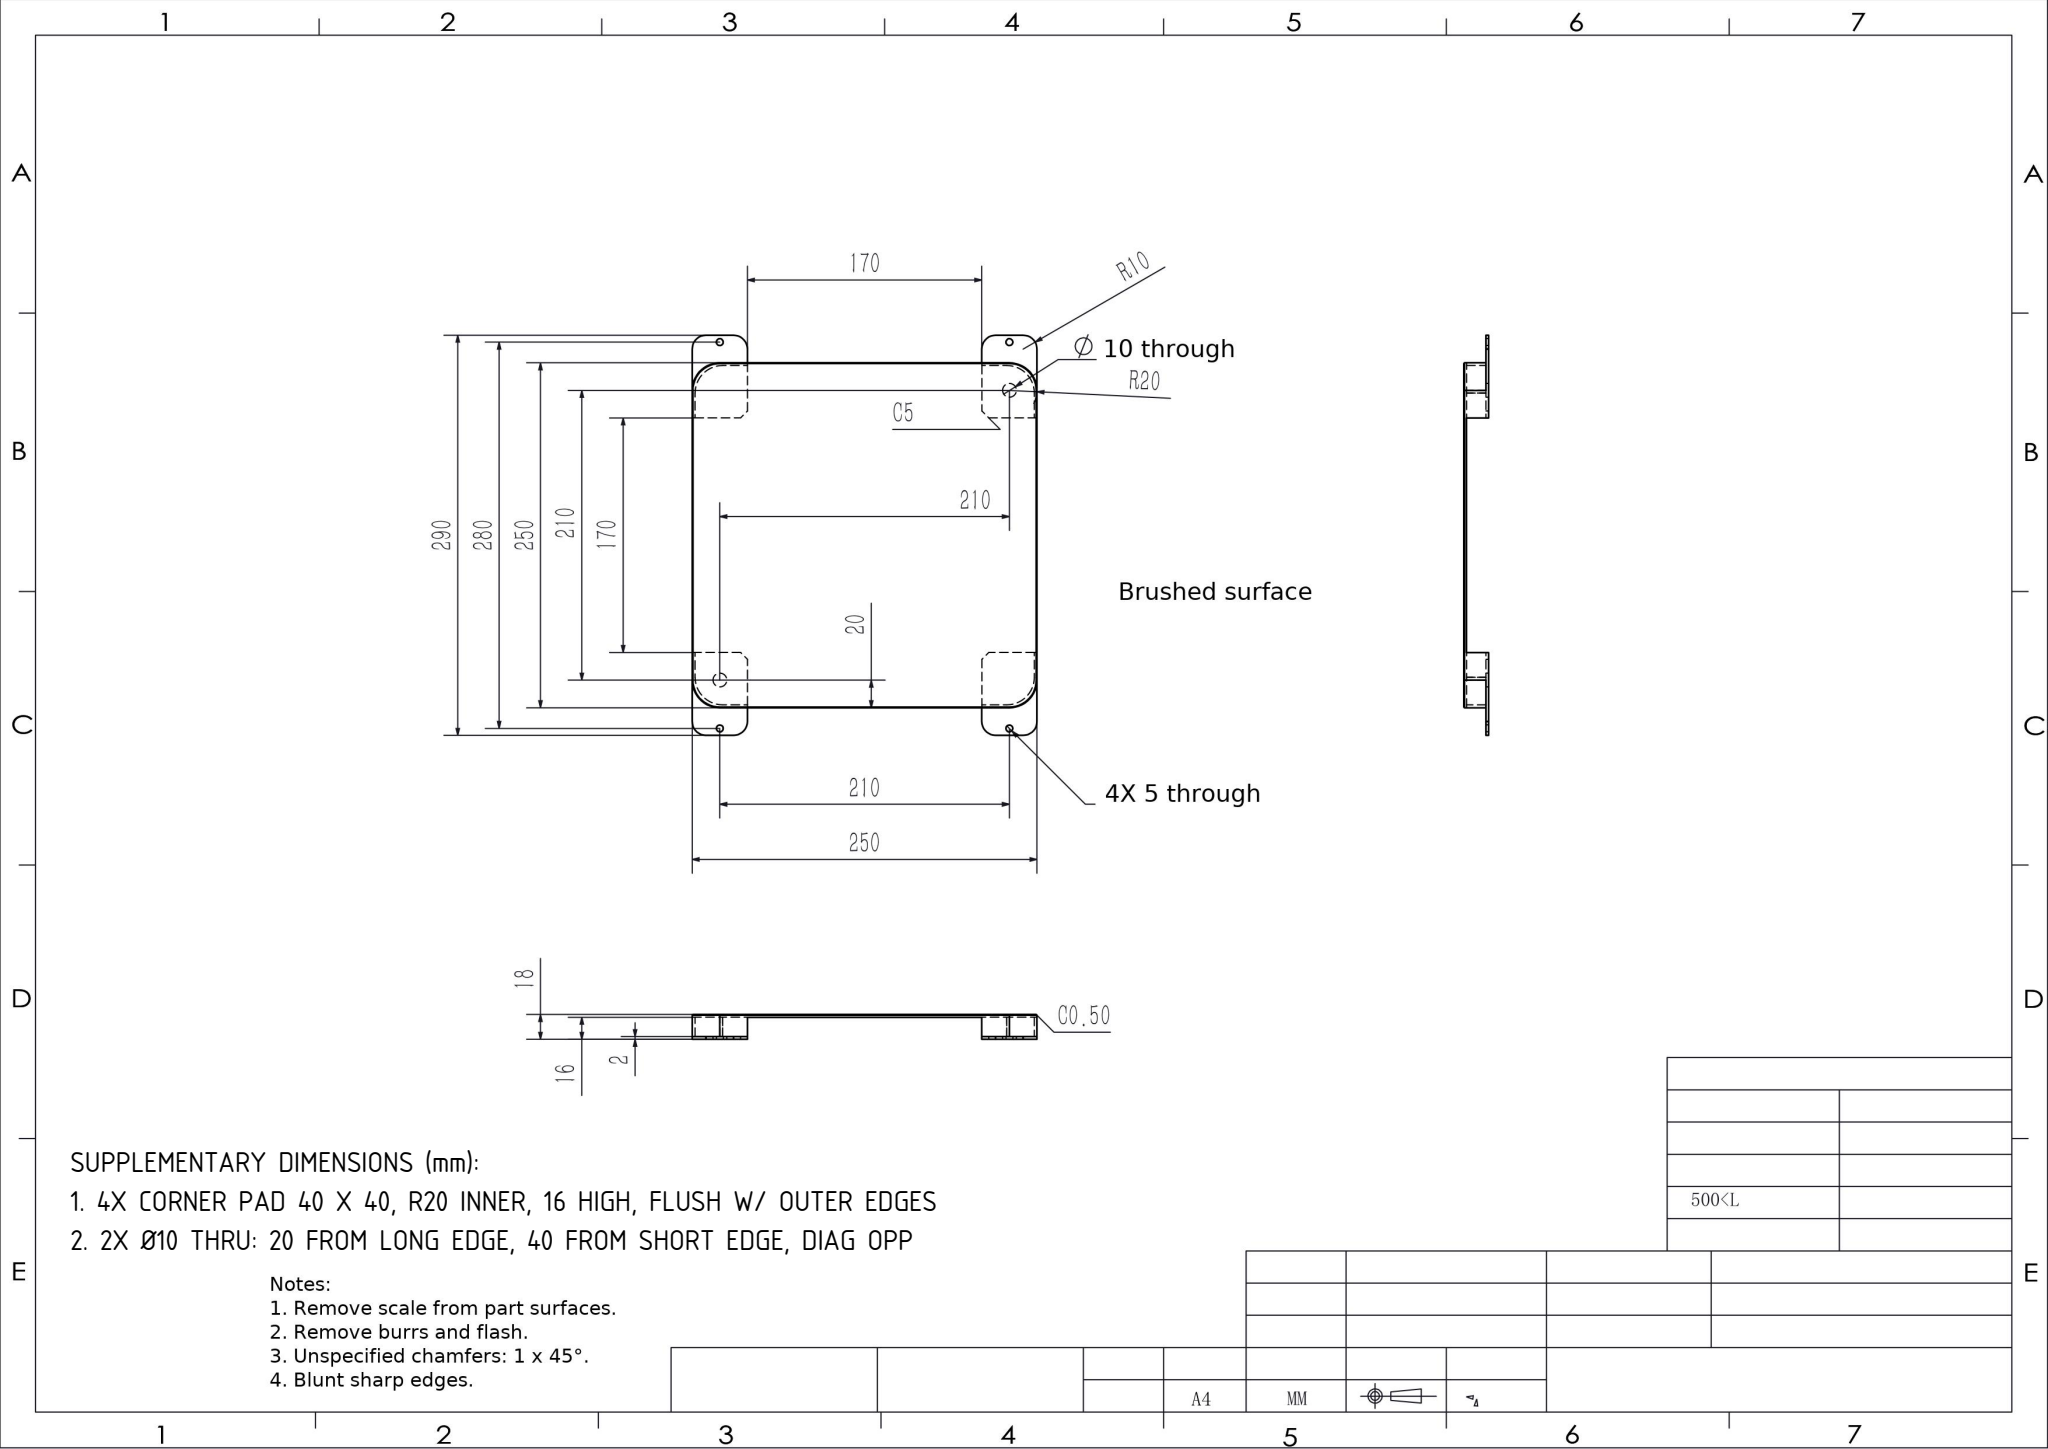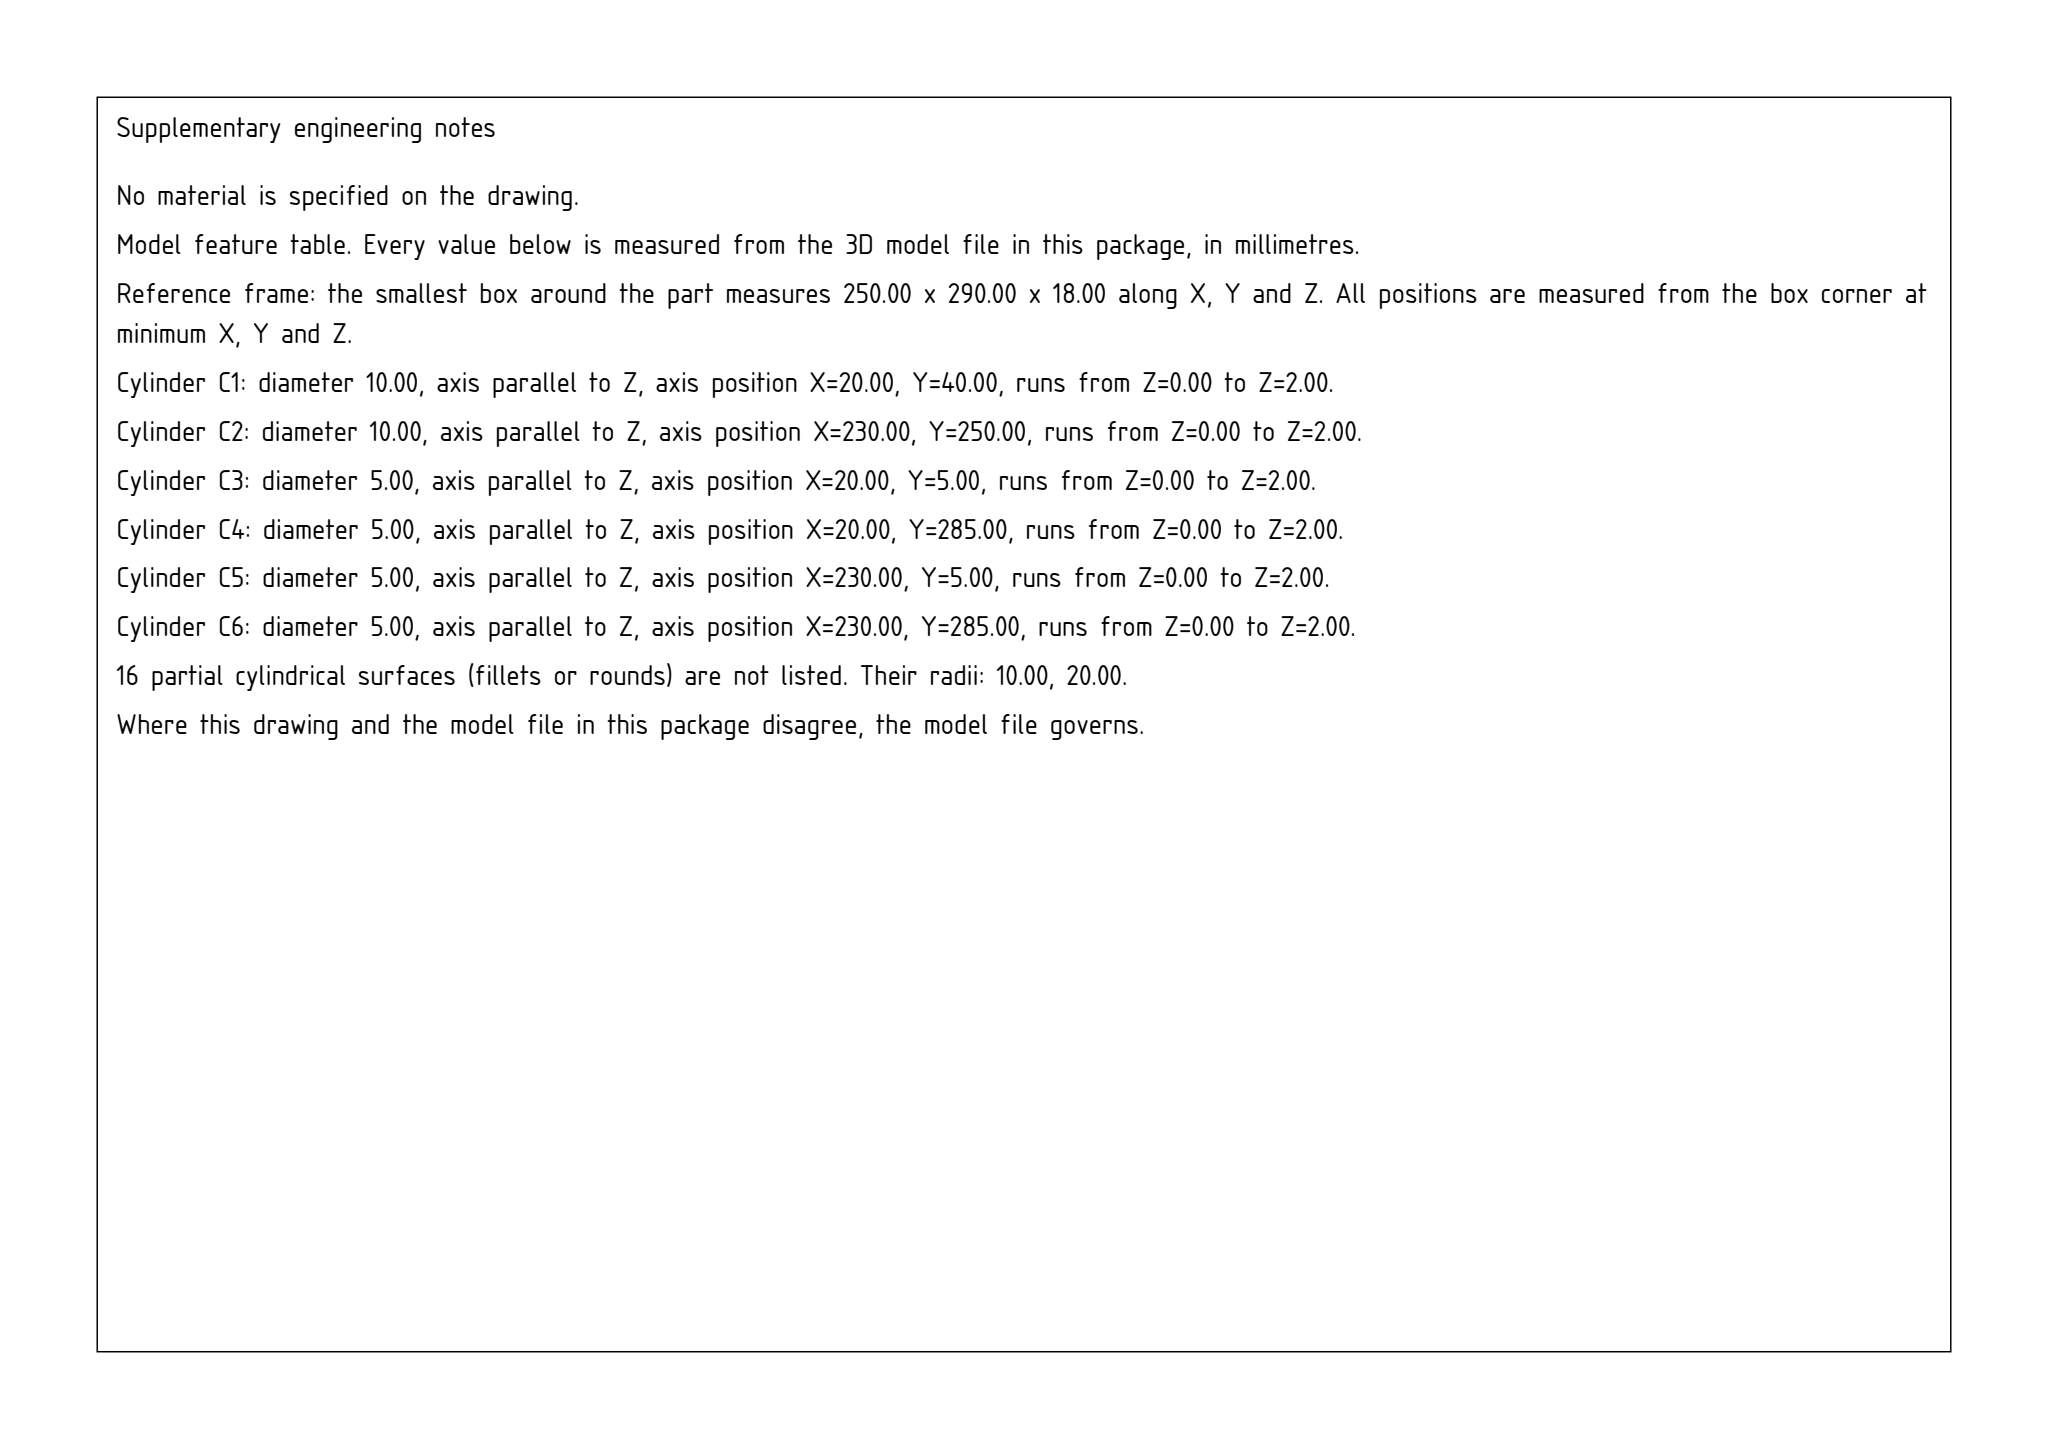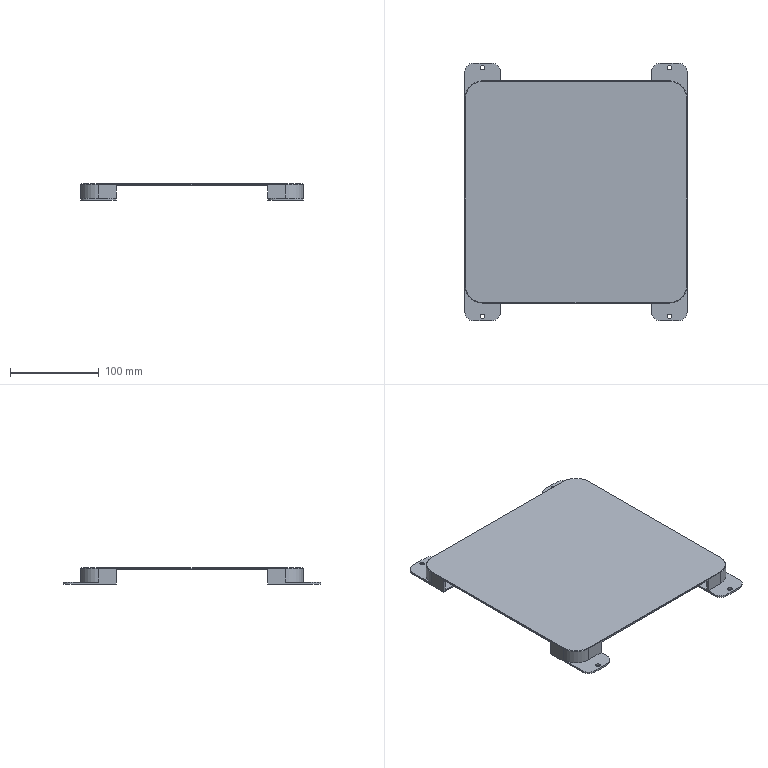Part | SolidWorks | mm | 1 solid | 78 faces | box 250 x 290 x 18 mm | volume 151214 mm3 | plane 46 | cylinder 28 | cone 4 | commonest cylinder face diameters 5 x8 40 x8 20 x8 10 x4
build123d program:
from build123d import *

# Parameters (mm, degrees)
SKETCH1_W           = 250
SKETCH1_H           = 250
BOSS_EXTRUDE1_DEPTH = 2
BOSS_EXTRUDE2_DEPTH = 14
SKETCH5_W           = 40
SKETCH5_H           = 40
BOSS_EXTRUDE3_DEPTH = 2
FILLET1_R           = 20
FILLET2_R           = 20
CHAMFER1_SIZE       = 0.5
CHAMFER2_SIZE       = 5
SKETCH6_R           = 5
CUT_EXTRUDE1_DEPTH  = 2
BOSS_EXTRUDE4_DEPTH = 2
FILLET3_R           = 10
SKETCH9_R           = 2.5
CUT_EXTRUDE2_DEPTH  = 193.109


with BuildPart() as part:
    # Sketch1 → Boss-Extrude1 (new body)
    with BuildSketch(Plane.XY):
        Rectangle(SKETCH1_W, SKETCH1_H)
    extrude(amount=BOSS_EXTRUDE1_DEPTH)

    # Sketch4 → Boss-Extrude2 (add)
    with BuildSketch(Plane(origin=(0, 0, 0), x_dir=(-1, 0, 0), z_dir=(0, 0, -1))):
        Polygon((85, 125), (125, 125), (125, 85), (123, 85), (123, 123), (85, 123), align=None)
        Polygon((-85, 123), (-123, 123), (-123, 85), (-125, 85), (-125, 125), (-85, 125), align=None)
        Polygon((-85, -125), (-125, -125), (-125, -85), (-123, -85), (-123, -123), (-85, -123), align=None)
        Polygon((85, -123), (123, -123), (123, -85), (125, -85), (125, -125), (85, -125), align=None)
    extrude(amount=BOSS_EXTRUDE2_DEPTH)

    # Sketch5 → Boss-Extrude3 (add)
    with BuildSketch(Plane(origin=(0, 0, -14), x_dir=(-1, 0, 0), z_dir=(0, 0, -1))):
        with Locations((105, 105)):
            Rectangle(SKETCH5_W, SKETCH5_H)
        with Locations((105, -105)):
            Rectangle(SKETCH5_W, SKETCH5_H)
        with Locations((-105, -105)):
            Rectangle(SKETCH5_W, SKETCH5_H)
        with Locations((-105, 105)):
            Rectangle(SKETCH5_W, SKETCH5_H)
    extrude(amount=BOSS_EXTRUDE3_DEPTH)

    # Fillet1
    fillet1_edges = [part.edges().sort_by_distance(p)[0] for p in [
        (125, -125, -7),
        (-125, -125, -7),
        (-125, 125, -7),
        (125, 125, -7),
    ]]
    fillet(fillet1_edges, radius=FILLET1_R)

    # Fillet2
    fillet2_edges = [part.edges().sort_by_distance(p)[0] for p in [
        (-123, 123, -7),
        (123, 123, -7),
        (123, -123, -7),
        (-123, -123, -7),
    ]]
    fillet(fillet2_edges, radius=FILLET2_R)

    # Chamfer1
    chamfer1_edges = [part.edges().sort_by_distance(p)[0] for p in [
        (-125, 0, 2),
        (0, 125, 2),
        (125, 0, 2),
        (0, -125, 2),
        (-119.142, -119.142, 2),
        (119.142, -119.142, 2),
        (119.142, 119.142, 2),
        (-119.142, 119.142, 2),
    ]]
    chamfer(chamfer1_edges, length=CHAMFER1_SIZE)

    # Chamfer2
    chamfer2_edges = [part.edges().sort_by_distance(p)[0] for p in [
        (85, -85, -15),
        (85, 85, -15),
        (-85, 85, -15),
        (-85, -85, -15),
    ]]
    chamfer(chamfer2_edges, length=CHAMFER2_SIZE)

    # Sketch6 → Cut-Extrude1 (cut)
    with BuildSketch(Plane(origin=(0, 0, -16), x_dir=(-1, 0, 0), z_dir=(0, 0, -1))):
        with Locations((-105, 105)):
            Circle(SKETCH6_R)
        with Locations((105, -105)):
            Circle(SKETCH6_R)
    extrude(amount=-CUT_EXTRUDE1_DEPTH, mode=Mode.SUBTRACT)

    # Sketch8 → Boss-Extrude4 (add)
    with BuildSketch(Plane(origin=(0, 0, -16), x_dir=(-1, 0, 0), z_dir=(0, 0, -1))):
        Polygon((-85, -100.761), (-95.852, -100.761), (-95.852, -116.476), (-113.788, -116.476), (-113.788, -100.761), (-125, -100.761), (-125, -145), (-85, -145), align=None)
        Polygon((-95.852, 100.761), (-95.852, 116.476), (-113.788, 116.476), (-113.788, 100.761), (-125, 100.761), (-125, 145), (-85, 145), (-85, 100.761), align=None)
        Polygon((95.852, -100.761), (95.852, -116.476), (113.788, -116.476), (113.788, -100.761), (125, -100.761), (125, -145), (85, -145), (85, -100.761), align=None)
        Polygon((85, 100.761), (95.852, 100.761), (95.852, 116.476), (113.788, 116.476), (113.788, 100.761), (125, 100.761), (125, 145), (85, 145), align=None)
    extrude(amount=-BOSS_EXTRUDE4_DEPTH)

    # Fillet3
    fillet3_edges = [part.edges().sort_by_distance(p)[0] for p in [
        (85, -145, -15),
        (125, -145, -15),
        (85, 145, -15),
        (125, 145, -15),
        (-85, -145, -15),
        (-125, -145, -15),
        (-85, 145, -15),
        (-125, 145, -15),
    ]]
    fillet(fillet3_edges, radius=FILLET3_R)

    # Sketch9 → Cut-Extrude2 (cut, through all)
    with BuildSketch(Plane.XY.offset(-14)):
        with Locations((-105, 140)):
            Circle(SKETCH9_R)
        with Locations(Location((105, 140, 0), (0, 0, 180))):
            Circle(SKETCH9_R)
        with Locations((105, -140)):
            Circle(SKETCH9_R)
        with Locations(Location((-105, -140, 0), (0, 0, 180))):
            Circle(SKETCH9_R)
    extrude(amount=-CUT_EXTRUDE2_DEPTH, mode=Mode.SUBTRACT)


solid = part.part